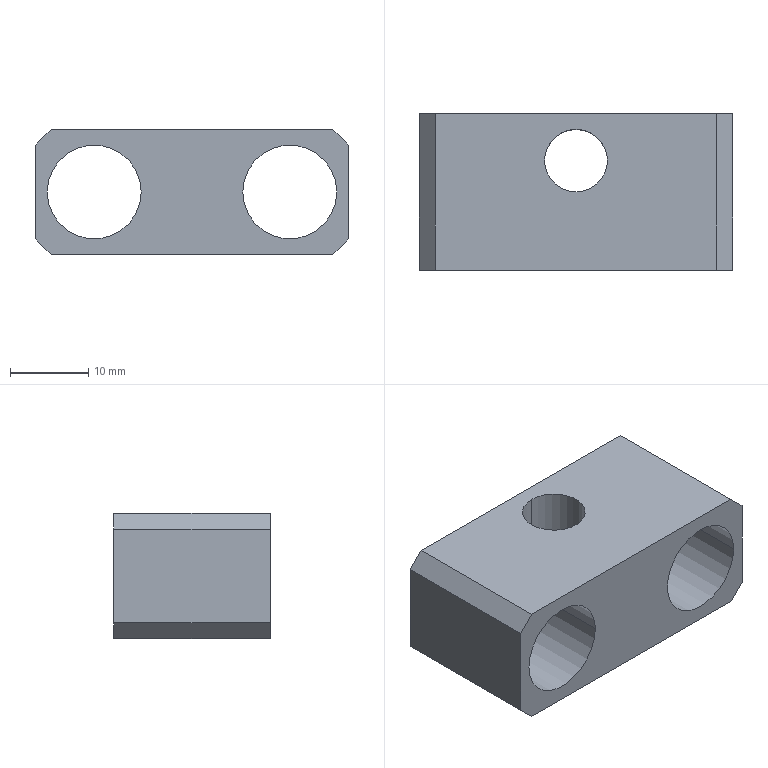Component | SolidWorks | GluePaperFeedingTensioningWheelAssembly-1_YX-04-117GluePaperFeedingTensioningWheelFixingPlate-1 | 1 solid | 19 faces | box 40 x 20 x 16 mm | volume 7216 mm3 | plane 11 | cylinder 8 | commonest cylinder face diameters 12 x4 9 x2 8 x2 | material 45#Steel
build123d program:
from build123d import *

# Parameters (mm, degrees)
SKETCH1_W                    = 40
SKETCH1_H                    = 20
BOSS_EXTRUDE1_DEPTH          = 16
F_8_0_8_DIAMETER_HOLE1_D     = 8
F_12_0_12_DIAMETER_HOLE1_D   = 12
F_12_0_12_DIAMETER_HOLE2_D   = 12
F_9_0_9_DIAMETER_HOLE1_D     = 9
F_9_0_9_DIAMETER_HOLE1_DEPTH = 1.5
CHAMFER1_SIZE                = 2


with BuildPart() as part:
    # Sketch1 → Boss-Extrude1 (new body)
    with BuildSketch(Plane(origin=(0, 8, 0), x_dir=(1, 0, 0), z_dir=(0, 1, 0))):
        Rectangle(SKETCH1_W, SKETCH1_H)
    extrude(amount=-BOSS_EXTRUDE1_DEPTH)

    # 8.0 _8_ Diameter Hole1 (through all)
    with Locations(Plane(origin=(0, -8, 0), x_dir=(-1, 0, 0), z_dir=(0, -1, 0))):
        with Locations((0, 4)):
            Hole(F_8_0_8_DIAMETER_HOLE1_D / 2)

    # 12.0 _12_ Diameter Hole1 (through all)
    with Locations(Plane(origin=(0, 0, -10), x_dir=(-1, 0, 0), z_dir=(0, 0, -1))):
        with Locations((12.5, 0)):
            Hole(F_12_0_12_DIAMETER_HOLE1_D / 2)

    # 12.0 _12_ Diameter Hole2 (through all)
    with Locations(Plane.XY.offset(10)):
        with Locations((12.5, 0)):
            Hole(F_12_0_12_DIAMETER_HOLE2_D / 2)

    # 9.0 _9_ Diameter Hole1
    with Locations(Plane(origin=(0, 0, -10), x_dir=(-1, 0, 0), z_dir=(0, 0, -1))):
        with Locations((0, 0)):
            Hole(F_9_0_9_DIAMETER_HOLE1_D / 2, depth=F_9_0_9_DIAMETER_HOLE1_DEPTH)

    # Chamfer1
    chamfer1_edges = [part.edges().sort_by_distance(p)[0] for p in [
        (-20, -8, 0),
        (20, -8, 0),
        (-20, 8, 0),
        (20, 8, 0),
    ]]
    chamfer(chamfer1_edges, length=CHAMFER1_SIZE)


solid = part.part

# Placed as in the assembly
solid = solid.moved(Location((16.603, 16.762, 167), (90, 0, 0)))
STEP:
#1=COLOUR_RGB('',0.7922,0.8196,0.9333);
#2=FILL_AREA_STYLE_COLOUR('',#1);
#3=FILL_AREA_STYLE('',(#2));
#4=SURFACE_STYLE_FILL_AREA(#3);
#5=SURFACE_SIDE_STYLE('',(#4));
#6=SURFACE_STYLE_USAGE(.BOTH.,#5);
#7=PRESENTATION_STYLE_ASSIGNMENT((#6));
#8=CARTESIAN_POINT('',(0.4765,0.9946,6.575));
#9=VERTEX_POINT('',#8);
#10=CARTESIAN_POINT('',(0.8308,0.9946,6.575));
#11=VERTEX_POINT('',#10);
#12=CARTESIAN_POINT('',(0.6537,0.9946,6.575));
#13=DIRECTION('',(-0.,1.,0.));
#14=DIRECTION('',(1.,0.,0.));
#15=AXIS2_PLACEMENT_3D('',#12,#13,#14);
#16=CIRCLE('',#15,0.1772);
#17=EDGE_CURVE('',#9,#11,#16,.T.);
#18=ORIENTED_EDGE('',*,*,#17,.F.);
#19=CARTESIAN_POINT('',(0.4765,1.054,6.575));
#20=VERTEX_POINT('',#19);
#21=CARTESIAN_POINT('',(0.4765,1.054,6.575));
#22=DIRECTION('',(-0.,1.,0.));
#23=VECTOR('',#22,39.37);
#24=LINE('',#21,#23);
#25=EDGE_CURVE('',#9,#20,#24,.T.);
#26=ORIENTED_EDGE('',*,*,#25,.T.);
#27=CARTESIAN_POINT('',(0.8308,1.054,6.575));
#28=VERTEX_POINT('',#27);
#29=CARTESIAN_POINT('',(0.6537,1.054,6.575));
#30=DIRECTION('',(-0.,1.,0.));
#31=DIRECTION('',(1.,0.,0.));
#32=AXIS2_PLACEMENT_3D('',#29,#30,#31);
#33=CIRCLE('',#32,0.1772);
#34=EDGE_CURVE('',#20,#28,#33,.T.);
#35=ORIENTED_EDGE('',*,*,#34,.T.);
#36=CARTESIAN_POINT('',(0.8308,1.054,6.575));
#37=DIRECTION('',(-0.,1.,0.));
#38=VECTOR('',#37,39.37);
#39=LINE('',#36,#38);
#40=EDGE_CURVE('',#11,#28,#39,.T.);
#41=ORIENTED_EDGE('',*,*,#40,.F.);
#42=EDGE_LOOP('',(#18,#26,#35,#41));
#43=FACE_OUTER_BOUND('',#42,.T.);
#44=CARTESIAN_POINT('',(0.6537,1.054,6.575));
#45=DIRECTION('',(-0.,1.,0.));
#46=DIRECTION('',(1.,0.,0.));
#47=AXIS2_PLACEMENT_3D('',#44,#45,#46);
#48=CYLINDRICAL_SURFACE('',#47,0.1772);
#49=ADVANCED_FACE('',(#43),#48,.F.);
#50=CARTESIAN_POINT('',(0.3977,1.054,6.575));
#51=VERTEX_POINT('',#50);
#52=CARTESIAN_POINT('',(-0.0747,1.054,6.575));
#53=VERTEX_POINT('',#52);
#54=CARTESIAN_POINT('',(0.1615,1.054,6.575));
#55=DIRECTION('',(0.,-1.,-0.));
#56=DIRECTION('',(-1.,0.,0.));
#57=AXIS2_PLACEMENT_3D('',#54,#55,#56);
#58=CIRCLE('',#57,0.2362);
#59=EDGE_CURVE('',#51,#53,#58,.T.);
#60=ORIENTED_EDGE('',*,*,#59,.F.);
#61=CARTESIAN_POINT('',(0.3977,0.2662,6.575));
#62=VERTEX_POINT('',#61);
#63=CARTESIAN_POINT('',(0.3977,0.2662,6.575));
#64=DIRECTION('',(0.,-1.,-0.));
#65=VECTOR('',#64,39.37);
#66=LINE('',#63,#65);
#67=EDGE_CURVE('',#51,#62,#66,.T.);
#68=ORIENTED_EDGE('',*,*,#67,.T.);
#69=CARTESIAN_POINT('',(-0.0747,0.2662,6.575));
#70=VERTEX_POINT('',#69);
#71=CARTESIAN_POINT('',(0.1615,0.2662,6.575));
#72=DIRECTION('',(0.,-1.,-0.));
#73=DIRECTION('',(-1.,0.,0.));
#74=AXIS2_PLACEMENT_3D('',#71,#72,#73);
#75=CIRCLE('',#74,0.2362);
#76=EDGE_CURVE('',#62,#70,#75,.T.);
#77=ORIENTED_EDGE('',*,*,#76,.T.);
#78=CARTESIAN_POINT('',(-0.0747,0.2662,6.575));
#79=DIRECTION('',(0.,-1.,-0.));
#80=VECTOR('',#79,39.37);
#81=LINE('',#78,#80);
#82=EDGE_CURVE('',#53,#70,#81,.T.);
#83=ORIENTED_EDGE('',*,*,#82,.F.);
#84=EDGE_LOOP('',(#60,#68,#77,#83));
#85=FACE_OUTER_BOUND('',#84,.T.);
#86=CARTESIAN_POINT('',(0.1615,0.2662,6.575));
#87=DIRECTION('',(0.,-1.,-0.));
#88=DIRECTION('',(-1.,0.,0.));
#89=AXIS2_PLACEMENT_3D('',#86,#87,#88);
#90=CYLINDRICAL_SURFACE('',#89,0.2362);
#91=ADVANCED_FACE('',(#85),#90,.F.);
#92=CARTESIAN_POINT('',(0.9096,0.2662,6.575));
#93=VERTEX_POINT('',#92);
#94=CARTESIAN_POINT('',(1.382,0.2662,6.575));
#95=VERTEX_POINT('',#94);
#96=CARTESIAN_POINT('',(1.146,0.2662,6.575));
#97=DIRECTION('',(-0.,1.,0.));
#98=DIRECTION('',(1.,0.,0.));
#99=AXIS2_PLACEMENT_3D('',#96,#97,#98);
#100=CIRCLE('',#99,0.2362);
#101=EDGE_CURVE('',#93,#95,#100,.T.);
#102=ORIENTED_EDGE('',*,*,#101,.F.);
#103=CARTESIAN_POINT('',(0.9096,1.054,6.575));
#104=VERTEX_POINT('',#103);
#105=CARTESIAN_POINT('',(0.9096,1.054,6.575));
#106=DIRECTION('',(-0.,1.,0.));
#107=VECTOR('',#106,39.37);
#108=LINE('',#105,#107);
#109=EDGE_CURVE('',#93,#104,#108,.T.);
#110=ORIENTED_EDGE('',*,*,#109,.T.);
#111=CARTESIAN_POINT('',(1.382,1.054,6.575));
#112=VERTEX_POINT('',#111);
#113=CARTESIAN_POINT('',(1.146,1.054,6.575));
#114=DIRECTION('',(-0.,1.,0.));
#115=DIRECTION('',(1.,0.,0.));
#116=AXIS2_PLACEMENT_3D('',#113,#114,#115);
#117=CIRCLE('',#116,0.2362);
#118=EDGE_CURVE('',#104,#112,#117,.T.);
#119=ORIENTED_EDGE('',*,*,#118,.T.);
#120=CARTESIAN_POINT('',(1.382,1.054,6.575));
#121=DIRECTION('',(-0.,1.,0.));
#122=VECTOR('',#121,39.37);
#123=LINE('',#120,#122);
#124=EDGE_CURVE('',#95,#112,#123,.T.);
#125=ORIENTED_EDGE('',*,*,#124,.F.);
#126=EDGE_LOOP('',(#102,#110,#119,#125));
#127=FACE_OUTER_BOUND('',#126,.T.);
#128=CARTESIAN_POINT('',(1.146,1.054,6.575));
#129=DIRECTION('',(-0.,1.,0.));
#130=DIRECTION('',(1.,0.,0.));
#131=AXIS2_PLACEMENT_3D('',#128,#129,#130);
#132=CYLINDRICAL_SURFACE('',#131,0.2362);
#133=ADVANCED_FACE('',(#127),#132,.F.);
#134=CARTESIAN_POINT('',(0.6537,0.6599,6.26));
#135=VERTEX_POINT('',#134);
#136=CARTESIAN_POINT('',(0.6537,0.9749,6.26));
#137=VERTEX_POINT('',#136);
#138=CARTESIAN_POINT('',(0.6537,0.8174,6.26));
#139=DIRECTION('',(-0.,-0.,1.));
#140=DIRECTION('',(0.,1.,0.));
#141=AXIS2_PLACEMENT_3D('',#138,#139,#140);
#142=CIRCLE('',#141,0.1575);
#143=EDGE_CURVE('',#135,#137,#142,.T.);
#144=ORIENTED_EDGE('',*,*,#143,.F.);
#145=CARTESIAN_POINT('',(0.6537,0.6599,6.89));
#146=VERTEX_POINT('',#145);
#147=CARTESIAN_POINT('',(0.6537,0.6599,6.89));
#148=DIRECTION('',(-0.,-0.,1.));
#149=VECTOR('',#148,39.37);
#150=LINE('',#147,#149);
#151=EDGE_CURVE('',#135,#146,#150,.T.);
#152=ORIENTED_EDGE('',*,*,#151,.T.);
#153=CARTESIAN_POINT('',(0.6537,0.9749,6.89));
#154=VERTEX_POINT('',#153);
#155=CARTESIAN_POINT('',(0.6537,0.8174,6.89));
#156=DIRECTION('',(-0.,-0.,1.));
#157=DIRECTION('',(0.,1.,0.));
#158=AXIS2_PLACEMENT_3D('',#155,#156,#157);
#159=CIRCLE('',#158,0.1575);
#160=EDGE_CURVE('',#146,#154,#159,.T.);
#161=ORIENTED_EDGE('',*,*,#160,.T.);
#162=CARTESIAN_POINT('',(0.6537,0.9749,6.89));
#163=DIRECTION('',(-0.,-0.,1.));
#164=VECTOR('',#163,39.37);
#165=LINE('',#162,#164);
#166=EDGE_CURVE('',#137,#154,#165,.T.);
#167=ORIENTED_EDGE('',*,*,#166,.F.);
#168=EDGE_LOOP('',(#144,#152,#161,#167));
#169=FACE_OUTER_BOUND('',#168,.T.);
#170=CARTESIAN_POINT('',(0.6537,0.8174,6.89));
#171=DIRECTION('',(-0.,-0.,1.));
#172=DIRECTION('',(0.,1.,0.));
#173=AXIS2_PLACEMENT_3D('',#170,#171,#172);
#174=CYLINDRICAL_SURFACE('',#173,0.1575);
#175=ADVANCED_FACE('',(#169),#174,.F.);
#176=CARTESIAN_POINT('',(-0.1338,0.2662,6.811));
#177=VERTEX_POINT('',#176);
#178=CARTESIAN_POINT('',(-0.1338,0.2662,6.339));
#179=VERTEX_POINT('',#178);
#180=CARTESIAN_POINT('',(-0.1338,0.2662,6.89));
#181=DIRECTION('',(0.,0.,-1.));
#182=VECTOR('',#181,39.37);
#183=LINE('',#180,#182);
#184=EDGE_CURVE('',#177,#179,#183,.T.);
#185=ORIENTED_EDGE('',*,*,#184,.F.);
#186=CARTESIAN_POINT('',(-0.1338,1.054,6.811));
#187=VERTEX_POINT('',#186);
#188=CARTESIAN_POINT('',(-0.1338,1.054,6.811));
#189=DIRECTION('',(-0.,1.,0.));
#190=VECTOR('',#189,39.37);
#191=LINE('',#188,#190);
#192=EDGE_CURVE('',#177,#187,#191,.T.);
#193=ORIENTED_EDGE('',*,*,#192,.T.);
#194=CARTESIAN_POINT('',(-0.1338,1.054,6.339));
#195=VERTEX_POINT('',#194);
#196=CARTESIAN_POINT('',(-0.1338,1.054,6.89));
#197=DIRECTION('',(0.,0.,-1.));
#198=VECTOR('',#197,39.37);
#199=LINE('',#196,#198);
#200=EDGE_CURVE('',#187,#195,#199,.T.);
#201=ORIENTED_EDGE('',*,*,#200,.T.);
#202=CARTESIAN_POINT('',(-0.1338,0.2662,6.339));
#203=DIRECTION('',(0.,-1.,-0.));
#204=VECTOR('',#203,39.37);
#205=LINE('',#202,#204);
#206=EDGE_CURVE('',#195,#179,#205,.T.);
#207=ORIENTED_EDGE('',*,*,#206,.T.);
#208=EDGE_LOOP('',(#185,#193,#201,#207));
#209=FACE_OUTER_BOUND('',#208,.T.);
#210=CARTESIAN_POINT('',(-0.1338,0.2662,6.89));
#211=DIRECTION('',(-1.,-0.,-0.));
#212=DIRECTION('',(-0.,1.,0.));
#213=AXIS2_PLACEMENT_3D('',#210,#211,#212);
#214=PLANE('',#213);
#215=ADVANCED_FACE('',(#209),#214,.T.);
#216=CARTESIAN_POINT('',(0.1615,0.2662,6.575));
#217=DIRECTION('',(0.,-1.,-0.));
#218=DIRECTION('',(-1.,0.,0.));
#219=AXIS2_PLACEMENT_3D('',#216,#217,#218);
#220=CIRCLE('',#219,0.2362);
#221=EDGE_CURVE('',#70,#62,#220,.T.);
#222=ORIENTED_EDGE('',*,*,#221,.F.);
#223=ORIENTED_EDGE('',*,*,#76,.F.);
#224=EDGE_LOOP('',(#222,#223));
#225=FACE_BOUND('',#224,.T.);
#226=CARTESIAN_POINT('',(1.146,0.2662,6.575));
#227=DIRECTION('',(-0.,1.,0.));
#228=DIRECTION('',(1.,0.,0.));
#229=AXIS2_PLACEMENT_3D('',#226,#227,#228);
#230=CIRCLE('',#229,0.2362);
#231=EDGE_CURVE('',#95,#93,#230,.T.);
#232=ORIENTED_EDGE('',*,*,#231,.T.);
#233=ORIENTED_EDGE('',*,*,#101,.T.);
#234=EDGE_LOOP('',(#232,#233));
#235=FACE_BOUND('',#234,.T.);
#236=CARTESIAN_POINT('',(1.441,0.2662,6.811));
#237=VERTEX_POINT('',#236);
#238=CARTESIAN_POINT('',(1.441,0.2662,6.339));
#239=VERTEX_POINT('',#238);
#240=CARTESIAN_POINT('',(1.441,0.2662,6.89));
#241=DIRECTION('',(0.,0.,-1.));
#242=VECTOR('',#241,39.37);
#243=LINE('',#240,#242);
#244=EDGE_CURVE('',#237,#239,#243,.T.);
#245=ORIENTED_EDGE('',*,*,#244,.F.);
#246=CARTESIAN_POINT('',(1.362,0.2662,6.89));
#247=VERTEX_POINT('',#246);
#248=CARTESIAN_POINT('',(1.402,0.2662,6.85));
#249=DIRECTION('',(-0.7071,-0.,0.7071));
#250=VECTOR('',#249,39.37);
#251=LINE('',#248,#250);
#252=EDGE_CURVE('',#237,#247,#251,.T.);
#253=ORIENTED_EDGE('',*,*,#252,.T.);
#254=CARTESIAN_POINT('',(-0.05501,0.2662,6.89));
#255=VERTEX_POINT('',#254);
#256=CARTESIAN_POINT('',(1.441,0.2662,6.89));
#257=DIRECTION('',(-1.,-0.,-0.));
#258=VECTOR('',#257,39.37);
#259=LINE('',#256,#258);
#260=EDGE_CURVE('',#247,#255,#259,.T.);
#261=ORIENTED_EDGE('',*,*,#260,.T.);
#262=CARTESIAN_POINT('',(0.693,0.2662,7.638));
#263=DIRECTION('',(-0.7071,-0.,-0.7071));
#264=VECTOR('',#263,39.37);
#265=LINE('',#262,#264);
#266=EDGE_CURVE('',#255,#177,#265,.T.);
#267=ORIENTED_EDGE('',*,*,#266,.T.);
#268=ORIENTED_EDGE('',*,*,#184,.T.);
#269=CARTESIAN_POINT('',(-0.05501,0.2662,6.26));
#270=VERTEX_POINT('',#269);
#271=CARTESIAN_POINT('',(0.3781,0.2662,5.827));
#272=DIRECTION('',(0.7071,0.,-0.7071));
#273=VECTOR('',#272,39.37);
#274=LINE('',#271,#273);
#275=EDGE_CURVE('',#179,#270,#274,.T.);
#276=ORIENTED_EDGE('',*,*,#275,.T.);
#277=CARTESIAN_POINT('',(1.362,0.2662,6.26));
#278=VERTEX_POINT('',#277);
#279=CARTESIAN_POINT('',(1.441,0.2662,6.26));
#280=DIRECTION('',(-1.,-0.,-0.));
#281=VECTOR('',#280,39.37);
#282=LINE('',#279,#281);
#283=EDGE_CURVE('',#278,#270,#282,.T.);
#284=ORIENTED_EDGE('',*,*,#283,.F.);
#285=CARTESIAN_POINT('',(1.717,0.2662,6.614));
#286=DIRECTION('',(0.7071,0.,0.7071));
#287=VECTOR('',#286,39.37);
#288=LINE('',#285,#287);
#289=EDGE_CURVE('',#278,#239,#288,.T.);
#290=ORIENTED_EDGE('',*,*,#289,.T.);
#291=EDGE_LOOP('',(#245,#253,#261,#267,#268,#276,#284,#290));
#292=FACE_OUTER_BOUND('',#291,.T.);
#293=CARTESIAN_POINT('',(1.441,0.2662,6.89));
#294=DIRECTION('',(0.,-1.,-0.));
#295=DIRECTION('',(-1.,-0.,-0.));
#296=AXIS2_PLACEMENT_3D('',#293,#294,#295);
#297=PLANE('',#296);
#298=ADVANCED_FACE('',(#225,#235,#292),#297,.T.);
#299=CARTESIAN_POINT('',(1.441,1.054,6.811));
#300=VERTEX_POINT('',#299);
#301=CARTESIAN_POINT('',(1.441,1.054,6.339));
#302=VERTEX_POINT('',#301);
#303=CARTESIAN_POINT('',(1.441,1.054,6.89));
#304=DIRECTION('',(0.,0.,-1.));
#305=VECTOR('',#304,39.37);
#306=LINE('',#303,#305);
#307=EDGE_CURVE('',#300,#302,#306,.T.);
#308=ORIENTED_EDGE('',*,*,#307,.F.);
#309=CARTESIAN_POINT('',(1.441,0.2662,6.811));
#310=DIRECTION('',(0.,-1.,-0.));
#311=VECTOR('',#310,39.37);
#312=LINE('',#309,#311);
#313=EDGE_CURVE('',#300,#237,#312,.T.);
#314=ORIENTED_EDGE('',*,*,#313,.T.);
#315=ORIENTED_EDGE('',*,*,#244,.T.);
#316=CARTESIAN_POINT('',(1.441,1.054,6.339));
#317=DIRECTION('',(-0.,1.,0.));
#318=VECTOR('',#317,39.37);
#319=LINE('',#316,#318);
#320=EDGE_CURVE('',#239,#302,#319,.T.);
#321=ORIENTED_EDGE('',*,*,#320,.T.);
#322=EDGE_LOOP('',(#308,#314,#315,#321));
#323=FACE_OUTER_BOUND('',#322,.T.);
#324=CARTESIAN_POINT('',(1.441,1.054,6.89));
#325=DIRECTION('',(1.,0.,0.));
#326=DIRECTION('',(0.,-1.,-0.));
#327=AXIS2_PLACEMENT_3D('',#324,#325,#326);
#328=PLANE('',#327);
#329=ADVANCED_FACE('',(#323),#328,.T.);
#330=CARTESIAN_POINT('',(0.6537,1.054,6.575));
#331=DIRECTION('',(-0.,1.,0.));
#332=DIRECTION('',(1.,0.,0.));
#333=AXIS2_PLACEMENT_3D('',#330,#331,#332);
#334=CIRCLE('',#333,0.1772);
#335=EDGE_CURVE('',#28,#20,#334,.T.);
#336=ORIENTED_EDGE('',*,*,#335,.F.);
#337=ORIENTED_EDGE('',*,*,#34,.F.);
#338=EDGE_LOOP('',(#336,#337));
#339=FACE_BOUND('',#338,.T.);
#340=CARTESIAN_POINT('',(0.1615,1.054,6.575));
#341=DIRECTION('',(0.,-1.,-0.));
#342=DIRECTION('',(-1.,0.,0.));
#343=AXIS2_PLACEMENT_3D('',#340,#341,#342);
#344=CIRCLE('',#343,0.2362);
#345=EDGE_CURVE('',#53,#51,#344,.T.);
#346=ORIENTED_EDGE('',*,*,#345,.T.);
#347=ORIENTED_EDGE('',*,*,#59,.T.);
#348=EDGE_LOOP('',(#346,#347));
#349=FACE_BOUND('',#348,.T.);
#350=CARTESIAN_POINT('',(1.146,1.054,6.575));
#351=DIRECTION('',(-0.,1.,0.));
#352=DIRECTION('',(1.,0.,0.));
#353=AXIS2_PLACEMENT_3D('',#350,#351,#352);
#354=CIRCLE('',#353,0.2362);
#355=EDGE_CURVE('',#112,#104,#354,.T.);
#356=ORIENTED_EDGE('',*,*,#355,.F.);
#357=ORIENTED_EDGE('',*,*,#118,.F.);
#358=EDGE_LOOP('',(#356,#357));
#359=FACE_BOUND('',#358,.T.);
#360=CARTESIAN_POINT('',(-0.05501,1.054,6.89));
#361=VERTEX_POINT('',#360);
#362=CARTESIAN_POINT('',(1.362,1.054,6.89));
#363=VERTEX_POINT('',#362);
#364=CARTESIAN_POINT('',(-0.1338,1.054,6.89));
#365=DIRECTION('',(1.,0.,0.));
#366=VECTOR('',#365,39.37);
#367=LINE('',#364,#366);
#368=EDGE_CURVE('',#361,#363,#367,.T.);
#369=ORIENTED_EDGE('',*,*,#368,.T.);
#370=CARTESIAN_POINT('',(0.6143,1.054,7.638));
#371=DIRECTION('',(0.7071,0.,-0.7071));
#372=VECTOR('',#371,39.37);
#373=LINE('',#370,#372);
#374=EDGE_CURVE('',#363,#300,#373,.T.);
#375=ORIENTED_EDGE('',*,*,#374,.T.);
#376=ORIENTED_EDGE('',*,*,#307,.T.);
#377=CARTESIAN_POINT('',(1.362,1.054,6.26));
#378=VERTEX_POINT('',#377);
#379=CARTESIAN_POINT('',(0.9292,1.054,5.827));
#380=DIRECTION('',(-0.7071,-0.,-0.7071));
#381=VECTOR('',#380,39.37);
#382=LINE('',#379,#381);
#383=EDGE_CURVE('',#302,#378,#382,.T.);
#384=ORIENTED_EDGE('',*,*,#383,.T.);
#385=CARTESIAN_POINT('',(-0.05501,1.054,6.26));
#386=VERTEX_POINT('',#385);
#387=CARTESIAN_POINT('',(-0.1338,1.054,6.26));
#388=DIRECTION('',(1.,0.,0.));
#389=VECTOR('',#388,39.37);
#390=LINE('',#387,#389);
#391=EDGE_CURVE('',#386,#378,#390,.T.);
#392=ORIENTED_EDGE('',*,*,#391,.F.);
#393=CARTESIAN_POINT('',(-0.4093,1.054,6.614));
#394=DIRECTION('',(-0.7071,-0.,0.7071));
#395=VECTOR('',#394,39.37);
#396=LINE('',#393,#395);
#397=EDGE_CURVE('',#386,#195,#396,.T.);
#398=ORIENTED_EDGE('',*,*,#397,.T.);
#399=ORIENTED_EDGE('',*,*,#200,.F.);
#400=CARTESIAN_POINT('',(-0.09438,1.054,6.85));
#401=DIRECTION('',(0.7071,0.,0.7071));
#402=VECTOR('',#401,39.37);
#403=LINE('',#400,#402);
#404=EDGE_CURVE('',#187,#361,#403,.T.);
#405=ORIENTED_EDGE('',*,*,#404,.T.);
#406=EDGE_LOOP('',(#369,#375,#376,#384,#392,#398,#399,#405));
#407=FACE_OUTER_BOUND('',#406,.T.);
#408=CARTESIAN_POINT('',(-0.1338,1.054,6.89));
#409=DIRECTION('',(-0.,1.,0.));
#410=DIRECTION('',(1.,0.,0.));
#411=AXIS2_PLACEMENT_3D('',#408,#409,#410);
#412=PLANE('',#411);
#413=ADVANCED_FACE('',(#339,#349,#359,#407),#412,.T.);
#414=CARTESIAN_POINT('',(0.6537,0.8174,6.89));
#415=DIRECTION('',(-0.,-0.,1.));
#416=DIRECTION('',(0.,1.,0.));
#417=AXIS2_PLACEMENT_3D('',#414,#415,#416);
#418=CIRCLE('',#417,0.1575);
#419=EDGE_CURVE('',#154,#146,#418,.T.);
#420=ORIENTED_EDGE('',*,*,#419,.F.);
#421=ORIENTED_EDGE('',*,*,#160,.F.);
#422=EDGE_LOOP('',(#420,#421));
#423=FACE_BOUND('',#422,.T.);
#424=ORIENTED_EDGE('',*,*,#260,.F.);
#425=CARTESIAN_POINT('',(1.362,1.054,6.89));
#426=DIRECTION('',(-0.,1.,0.));
#427=VECTOR('',#426,39.37);
#428=LINE('',#425,#427);
#429=EDGE_CURVE('',#247,#363,#428,.T.);
#430=ORIENTED_EDGE('',*,*,#429,.T.);
#431=ORIENTED_EDGE('',*,*,#368,.F.);
#432=CARTESIAN_POINT('',(-0.05501,0.2662,6.89));
#433=DIRECTION('',(0.,-1.,-0.));
#434=VECTOR('',#433,39.37);
#435=LINE('',#432,#434);
#436=EDGE_CURVE('',#361,#255,#435,.T.);
#437=ORIENTED_EDGE('',*,*,#436,.T.);
#438=EDGE_LOOP('',(#424,#430,#431,#437));
#439=FACE_OUTER_BOUND('',#438,.T.);
#440=CARTESIAN_POINT('',(0.6537,0.6599,6.89));
#441=DIRECTION('',(0.,0.,-1.));
#442=DIRECTION('',(0.,-1.,-0.));
#443=AXIS2_PLACEMENT_3D('',#440,#441,#442);
#444=PLANE('',#443);
#445=ADVANCED_FACE('',(#423,#439),#444,.F.);
#446=CARTESIAN_POINT('',(0.6537,0.8174,6.26));
#447=DIRECTION('',(-0.,-0.,1.));
#448=DIRECTION('',(0.,1.,0.));
#449=AXIS2_PLACEMENT_3D('',#446,#447,#448);
#450=CIRCLE('',#449,0.1575);
#451=EDGE_CURVE('',#137,#135,#450,.T.);
#452=ORIENTED_EDGE('',*,*,#451,.T.);
#453=ORIENTED_EDGE('',*,*,#143,.T.);
#454=EDGE_LOOP('',(#452,#453));
#455=FACE_BOUND('',#454,.T.);
#456=ORIENTED_EDGE('',*,*,#283,.T.);
#457=CARTESIAN_POINT('',(-0.05501,0.6599,6.26));
#458=DIRECTION('',(-0.,1.,0.));
#459=VECTOR('',#458,39.37);
#460=LINE('',#457,#459);
#461=EDGE_CURVE('',#270,#386,#460,.T.);
#462=ORIENTED_EDGE('',*,*,#461,.T.);
#463=ORIENTED_EDGE('',*,*,#391,.T.);
#464=CARTESIAN_POINT('',(1.362,0.6599,6.26));
#465=DIRECTION('',(0.,-1.,-0.));
#466=VECTOR('',#465,39.37);
#467=LINE('',#464,#466);
#468=EDGE_CURVE('',#378,#278,#467,.T.);
#469=ORIENTED_EDGE('',*,*,#468,.T.);
#470=EDGE_LOOP('',(#456,#462,#463,#469));
#471=FACE_OUTER_BOUND('',#470,.T.);
#472=CARTESIAN_POINT('',(0.6537,0.6599,6.26));
#473=DIRECTION('',(0.,0.,-1.));
#474=DIRECTION('',(0.,-1.,-0.));
#475=AXIS2_PLACEMENT_3D('',#472,#473,#474);
#476=PLANE('',#475);
#477=ADVANCED_FACE('',(#455,#471),#476,.T.);
#478=ORIENTED_EDGE('',*,*,#151,.F.);
#479=ORIENTED_EDGE('',*,*,#451,.F.);
#480=ORIENTED_EDGE('',*,*,#166,.T.);
#481=ORIENTED_EDGE('',*,*,#419,.T.);
#482=EDGE_LOOP('',(#478,#479,#480,#481));
#483=FACE_OUTER_BOUND('',#482,.T.);
#484=CARTESIAN_POINT('',(0.6537,0.8174,6.89));
#485=DIRECTION('',(-0.,-0.,1.));
#486=DIRECTION('',(0.,1.,0.));
#487=AXIS2_PLACEMENT_3D('',#484,#485,#486);
#488=CYLINDRICAL_SURFACE('',#487,0.1575);
#489=ADVANCED_FACE('',(#483),#488,.F.);
#490=ORIENTED_EDGE('',*,*,#109,.F.);
#491=ORIENTED_EDGE('',*,*,#231,.F.);
#492=ORIENTED_EDGE('',*,*,#124,.T.);
#493=ORIENTED_EDGE('',*,*,#355,.T.);
#494=EDGE_LOOP('',(#490,#491,#492,#493));
#495=FACE_OUTER_BOUND('',#494,.T.);
#496=CARTESIAN_POINT('',(1.146,1.054,6.575));
#497=DIRECTION('',(-0.,1.,0.));
#498=DIRECTION('',(1.,0.,0.));
#499=AXIS2_PLACEMENT_3D('',#496,#497,#498);
#500=CYLINDRICAL_SURFACE('',#499,0.2362);
#501=ADVANCED_FACE('',(#495),#500,.F.);
#502=ORIENTED_EDGE('',*,*,#67,.F.);
#503=ORIENTED_EDGE('',*,*,#345,.F.);
#504=ORIENTED_EDGE('',*,*,#82,.T.);
#505=ORIENTED_EDGE('',*,*,#221,.T.);
#506=EDGE_LOOP('',(#502,#503,#504,#505));
#507=FACE_OUTER_BOUND('',#506,.T.);
#508=CARTESIAN_POINT('',(0.1615,0.2662,6.575));
#509=DIRECTION('',(0.,-1.,-0.));
#510=DIRECTION('',(-1.,0.,0.));
#511=AXIS2_PLACEMENT_3D('',#508,#509,#510);
#512=CYLINDRICAL_SURFACE('',#511,0.2362);
#513=ADVANCED_FACE('',(#507),#512,.F.);
#514=CARTESIAN_POINT('',(0.6537,0.9946,6.575));
#515=DIRECTION('',(-0.,1.,0.));
#516=DIRECTION('',(1.,0.,0.));
#517=AXIS2_PLACEMENT_3D('',#514,#515,#516);
#518=CIRCLE('',#517,0.1772);
#519=EDGE_CURVE('',#11,#9,#518,.T.);
#520=ORIENTED_EDGE('',*,*,#519,.T.);
#521=ORIENTED_EDGE('',*,*,#17,.T.);
#522=EDGE_LOOP('',(#520,#521));
#523=FACE_OUTER_BOUND('',#522,.T.);
#524=CARTESIAN_POINT('',(0.6537,0.9946,6.575));
#525=DIRECTION('',(0.,-1.,-0.));
#526=DIRECTION('',(-1.,-0.,-0.));
#527=AXIS2_PLACEMENT_3D('',#524,#525,#526);
#528=PLANE('',#527);
#529=ADVANCED_FACE('',(#523),#528,.F.);
#530=ORIENTED_EDGE('',*,*,#25,.F.);
#531=ORIENTED_EDGE('',*,*,#519,.F.);
#532=ORIENTED_EDGE('',*,*,#40,.T.);
#533=ORIENTED_EDGE('',*,*,#335,.T.);
#534=EDGE_LOOP('',(#530,#531,#532,#533));
#535=FACE_OUTER_BOUND('',#534,.T.);
#536=CARTESIAN_POINT('',(0.6537,1.054,6.575));
#537=DIRECTION('',(-0.,1.,0.));
#538=DIRECTION('',(1.,0.,0.));
#539=AXIS2_PLACEMENT_3D('',#536,#537,#538);
#540=CYLINDRICAL_SURFACE('',#539,0.1772);
#541=ADVANCED_FACE('',(#535),#540,.F.);
#542=ORIENTED_EDGE('',*,*,#374,.F.);
#543=ORIENTED_EDGE('',*,*,#429,.F.);
#544=ORIENTED_EDGE('',*,*,#252,.F.);
#545=ORIENTED_EDGE('',*,*,#313,.F.);
#546=EDGE_LOOP('',(#542,#543,#544,#545));
#547=FACE_OUTER_BOUND('',#546,.T.);
#548=CARTESIAN_POINT('',(1.441,1.054,6.811));
#549=DIRECTION('',(0.7071,-0.,0.7071));
#550=DIRECTION('',(-0.,1.,0.));
#551=AXIS2_PLACEMENT_3D('',#548,#549,#550);
#552=PLANE('',#551);
#553=ADVANCED_FACE('',(#547),#552,.T.);
#554=ORIENTED_EDGE('',*,*,#266,.F.);
#555=ORIENTED_EDGE('',*,*,#436,.F.);
#556=ORIENTED_EDGE('',*,*,#404,.F.);
#557=ORIENTED_EDGE('',*,*,#192,.F.);
#558=EDGE_LOOP('',(#554,#555,#556,#557));
#559=FACE_OUTER_BOUND('',#558,.T.);
#560=CARTESIAN_POINT('',(-0.1338,0.2662,6.811));
#561=DIRECTION('',(-0.7071,-0.,0.7071));
#562=DIRECTION('',(0.,-1.,-0.));
#563=AXIS2_PLACEMENT_3D('',#560,#561,#562);
#564=PLANE('',#563);
#565=ADVANCED_FACE('',(#559),#564,.T.);
#566=ORIENTED_EDGE('',*,*,#275,.F.);
#567=ORIENTED_EDGE('',*,*,#206,.F.);
#568=ORIENTED_EDGE('',*,*,#397,.F.);
#569=ORIENTED_EDGE('',*,*,#461,.F.);
#570=EDGE_LOOP('',(#566,#567,#568,#569));
#571=FACE_OUTER_BOUND('',#570,.T.);
#572=CARTESIAN_POINT('',(-0.05501,0.6599,6.26));
#573=DIRECTION('',(0.7071,0.,0.7071));
#574=DIRECTION('',(-0.,1.,0.));
#575=AXIS2_PLACEMENT_3D('',#572,#573,#574);
#576=PLANE('',#575);
#577=ADVANCED_FACE('',(#571),#576,.F.);
#578=ORIENTED_EDGE('',*,*,#383,.F.);
#579=ORIENTED_EDGE('',*,*,#320,.F.);
#580=ORIENTED_EDGE('',*,*,#289,.F.);
#581=ORIENTED_EDGE('',*,*,#468,.F.);
#582=EDGE_LOOP('',(#578,#579,#580,#581));
#583=FACE_OUTER_BOUND('',#582,.T.);
#584=CARTESIAN_POINT('',(1.362,0.6599,6.26));
#585=DIRECTION('',(-0.7071,-0.,0.7071));
#586=DIRECTION('',(0.,-1.,-0.));
#587=AXIS2_PLACEMENT_3D('',#584,#585,#586);
#588=PLANE('',#587);
#589=ADVANCED_FACE('',(#583),#588,.F.);
#590=CLOSED_SHELL('',(#49,#91,#133,#175,#215,#298,#329,#413,#445,#477,#489,#501,#513,#529,#541,#553,#565,#577,#589));
#591=MANIFOLD_SOLID_BREP('',#590);
#592=STYLED_ITEM('',(#7),#591);
#593=PRESENTATION_LAYER_ASSIGNMENT('','',(#592));
#594=(LENGTH_UNIT()NAMED_UNIT(*)SI_UNIT($,.METRE.));
#595=LENGTH_MEASURE_WITH_UNIT(LENGTH_MEASURE(0.0254),#594);
#596=DIMENSIONAL_EXPONENTS(1.,0.,0.,0.,0.,0.,0.);
#597=(CONVERSION_BASED_UNIT('',#595)LENGTH_UNIT()NAMED_UNIT(#596));
#598=UNCERTAINTY_MEASURE_WITH_UNIT(LENGTH_MEASURE(0.00001),#597,'','');
#599=(NAMED_UNIT(*)PLANE_ANGLE_UNIT()SI_UNIT($,.RADIAN.));
#600=(NAMED_UNIT(*)SI_UNIT($,.STERADIAN.)SOLID_ANGLE_UNIT());
#601=(GEOMETRIC_REPRESENTATION_CONTEXT(3)GLOBAL_UNCERTAINTY_ASSIGNED_CONTEXT((#598))GLOBAL_UNIT_ASSIGNED_CONTEXT((#597,#599,#600))REPRESENTATION_CONTEXT('',''));
#602=MECHANICAL_DESIGN_GEOMETRIC_PRESENTATION_REPRESENTATION('',(#592),#601);
#603=CARTESIAN_POINT('',(0.,0.,0.));
#604=DIRECTION('',(0.,0.,1.));
#605=DIRECTION('',(1.,0.,0.));
#606=AXIS2_PLACEMENT_3D('',#603,#604,#605);
#607=(LENGTH_UNIT()NAMED_UNIT(*)SI_UNIT($,.METRE.));
#608=LENGTH_MEASURE_WITH_UNIT(LENGTH_MEASURE(0.0254),#607);
#609=DIMENSIONAL_EXPONENTS(1.,0.,0.,0.,0.,0.,0.);
#610=(CONVERSION_BASED_UNIT('',#608)LENGTH_UNIT()NAMED_UNIT(#609));
#611=UNCERTAINTY_MEASURE_WITH_UNIT(LENGTH_MEASURE(0.00001),#610,'','');
#612=(NAMED_UNIT(*)PLANE_ANGLE_UNIT()SI_UNIT($,.RADIAN.));
#613=(NAMED_UNIT(*)SI_UNIT($,.STERADIAN.)SOLID_ANGLE_UNIT());
#614=(GEOMETRIC_REPRESENTATION_CONTEXT(3)GLOBAL_UNCERTAINTY_ASSIGNED_CONTEXT((#611))GLOBAL_UNIT_ASSIGNED_CONTEXT((#610,#612,#613))REPRESENTATION_CONTEXT('',''));
#615=ADVANCED_BREP_SHAPE_REPRESENTATION('',(#591,#606),#614);